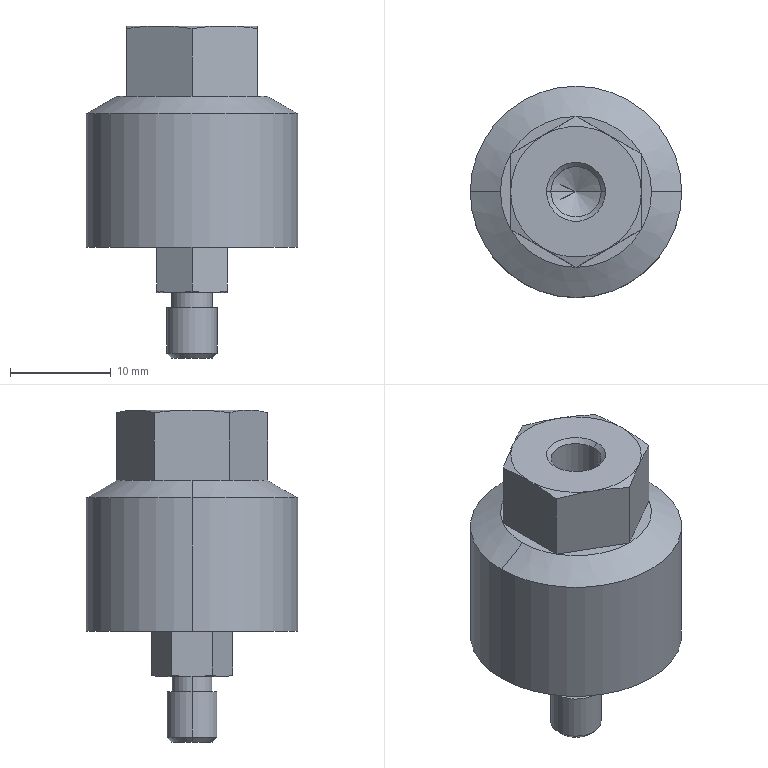Component | SolidWorks | F-YBJB20-5-080(0)-1 | 1 solid | 51 faces | box 21 x 21 x 33 mm | volume 6202 mm3 | plane 23 | cone 20 | cylinder 8 | commonest cylinder face diameters 5 x4 4 x2 21 x2
build123d program:
from build123d import *

# Parameters (mm, degrees)
SKETCH2_R          = 8.45
CUT_EXTRUDE1_DEPTH = 7
SKETCH3_R          = 4.55
CUT_EXTRUDE2_DEPTH = 4.5
HOLE1_D            = 5
HOLE1_DEPTH        = 8
HOLE1_CSINK_D      = 5.866
HOLE1_CSINK_ANGLE  = 90
HOLE1_TIP          = 1.443


with BuildPart() as part:
    # Sketch1 → Revolve1 (revolve)
    with BuildSketch(Plane.XY, mode=Mode.PRIVATE) as revolve1_sk:
        Polygon((-33, 0), (-33, 2.01), (-32.51, 2.5), (-28, 2.5), (-28, 2), (-26.5, 2), (-26.5, 3.5), (-26.312, 4.2), (-22, 4.2), (-22, 10.5), (-8.729, 10.5), (-7, 7.506), (-0.2694, 7.506), (0, 6.5), (0, 0), align=None)
    revolve(revolve1_sk.sketch.rotate(Axis((0, 0, 0), (-1, 0, 0)), 270), axis=Axis((0, 0, 0), (-1, 0, 0)))

    # Sketch2 → Cut-Extrude1 (cut)
    with BuildSketch(Plane(origin=(0, 0, 0), x_dir=(0, 0, -1), z_dir=(1, 0, 0))):
        Circle(SKETCH2_R)
        Polygon((-6.5, 3.753), (-6.5, -3.753), (0, -7.506), (6.5, -3.753), (6.5, 3.753), (0, 7.506), align=None, mode=Mode.SUBTRACT)
    extrude(amount=-CUT_EXTRUDE1_DEPTH, mode=Mode.SUBTRACT)

    # Sketch3 → Cut-Extrude2 (cut)
    with BuildSketch(Plane(origin=(-26.5, 0, 0), x_dir=(0, 0, -1), z_dir=(1, 0, 0))):
        Circle(SKETCH3_R)
        Polygon((-3.5, 2.021), (-3.5, -2.021), (0, -4.041), (3.5, -2.021), (3.5, 2.021), (0, 4.041), align=None, mode=Mode.SUBTRACT)
    extrude(amount=CUT_EXTRUDE2_DEPTH, mode=Mode.SUBTRACT)

    # Hole1
    with Locations(Plane(origin=(0, 0, 0), x_dir=(0, 0, -1), z_dir=(1, 0, 0))):
        with Locations((0, 0)):
            CounterSinkHole(HOLE1_D / 2, HOLE1_CSINK_D / 2, depth=HOLE1_DEPTH, counter_sink_angle=HOLE1_CSINK_ANGLE)
            with Locations((0, 0, -(HOLE1_DEPTH + HOLE1_TIP / 2))):  # 120° drill point
                Cone(0, HOLE1_D / 2, HOLE1_TIP, mode=Mode.SUBTRACT)


solid = part.part

# Placed as in the assembly
solid = solid.moved(Location((272.305, 302.175, 112.479), (0, -90, 0)))